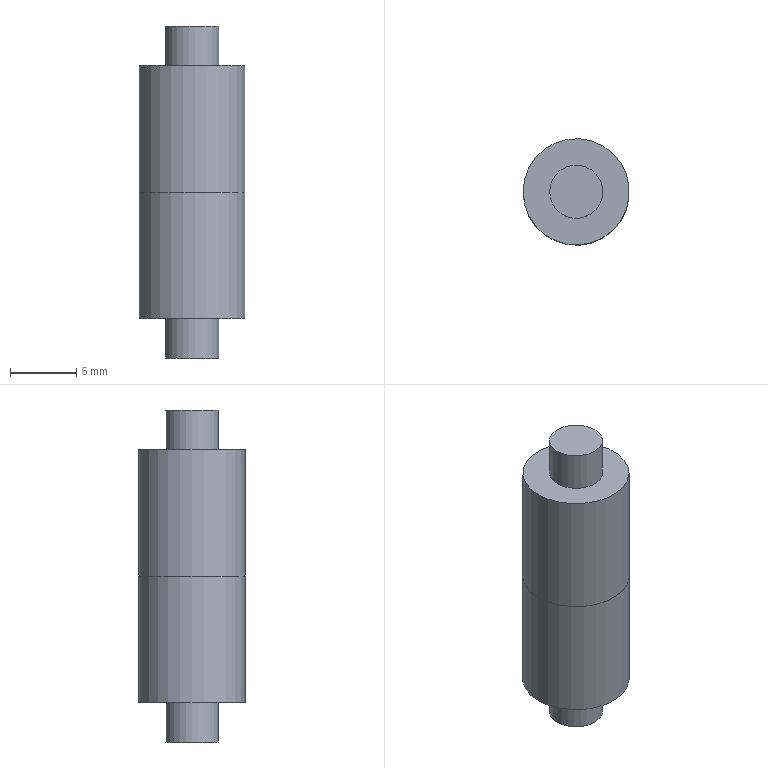Component | NX | MODEL5 | 2 solids | 10 faces | box 8 x 8 x 25 mm | volume 1030 mm3 | plane 6 | cylinder 4 | commonest cylinder face diameters 8 x2 4 x2
STEP:
#1=CARTESIAN_POINT('',(0.,0.,0.));
#2=DIRECTION('',(0.,0.,1.));
#3=DIRECTION('',(1.,0.,0.));
#4=AXIS2_PLACEMENT_3D('',#1,#2,#3);
#5=CARTESIAN_POINT('',(-1.53,2.589,6.));
#6=VERTEX_POINT('',#5);
#7=CARTESIAN_POINT('',(2.47,2.589,6.));
#8=DIRECTION('',(0.,0.,-1.));
#9=DIRECTION('',(-1.,0.,0.));
#10=AXIS2_PLACEMENT_3D('',#7,#8,#9);
#11=CIRCLE('',#10,4.);
#12=CARTESIAN_POINT('',(2.47,4.589,6.));
#13=DIRECTION('',(0.,0.,-1.));
#14=DIRECTION('',(-1.,0.,0.));
#15=AXIS2_PLACEMENT_3D('',#12,#13,#14);
#16=PLANE('',#15);
#17=CARTESIAN_POINT('',(0.,-2.));
#18=DIRECTION('',(1.,0.));
#19=AXIS2_PLACEMENT_2D('',#17,#18);
#20=CIRCLE('',#19,4.);
#21=(GEOMETRIC_REPRESENTATION_CONTEXT(2)PARAMETRIC_REPRESENTATION_CONTEXT()REPRESENTATION_CONTEXT('',''));
#22=DEFINITIONAL_REPRESENTATION('',(#20),#21);
#23=PCURVE('',#16,#22);
#24=CARTESIAN_POINT('',(2.47,2.589,3.));
#25=DIRECTION('',(0.,0.,-1.));
#26=DIRECTION('',(-1.,0.,0.));
#27=AXIS2_PLACEMENT_3D('',#24,#25,#26);
#28=CYLINDRICAL_SURFACE('',#27,4.);
#29=CARTESIAN_POINT('',(0.,-3.));
#30=DIRECTION('',(1.,0.));
#31=VECTOR('',#30,1.);
#32=LINE('',#29,#31);
#33=(GEOMETRIC_REPRESENTATION_CONTEXT(2)PARAMETRIC_REPRESENTATION_CONTEXT()REPRESENTATION_CONTEXT('',''));
#34=DEFINITIONAL_REPRESENTATION('',(#32),#33);
#35=PCURVE('',#28,#34);
#36=SURFACE_CURVE('',#11,(#23,#35),.PCURVE_S1.);
#37=EDGE_CURVE('',#6,#6,#36,.T.);
#38=ORIENTED_EDGE('',*,*,#37,.T.);
#39=EDGE_LOOP('',(#38));
#40=FACE_BOUND('',#39,.T.);
#41=CARTESIAN_POINT('',(0.4703,2.589,6.));
#42=VERTEX_POINT('',#41);
#43=CARTESIAN_POINT('',(2.47,2.589,6.));
#44=DIRECTION('',(0.,0.,-1.));
#45=DIRECTION('',(-1.,0.,0.));
#46=AXIS2_PLACEMENT_3D('',#43,#44,#45);
#47=CIRCLE('',#46,2.);
#48=CARTESIAN_POINT('',(0.,-2.));
#49=DIRECTION('',(1.,0.));
#50=AXIS2_PLACEMENT_2D('',#48,#49);
#51=CIRCLE('',#50,2.);
#52=(GEOMETRIC_REPRESENTATION_CONTEXT(2)PARAMETRIC_REPRESENTATION_CONTEXT()REPRESENTATION_CONTEXT('',''));
#53=DEFINITIONAL_REPRESENTATION('',(#51),#52);
#54=PCURVE('',#16,#53);
#55=CARTESIAN_POINT('',(2.47,2.589,3.));
#56=DIRECTION('',(0.,0.,-1.));
#57=DIRECTION('',(-1.,0.,0.));
#58=AXIS2_PLACEMENT_3D('',#55,#56,#57);
#59=CYLINDRICAL_SURFACE('',#58,2.);
#60=CARTESIAN_POINT('',(0.,-3.));
#61=DIRECTION('',(1.,0.));
#62=VECTOR('',#61,1.);
#63=LINE('',#60,#62);
#64=(GEOMETRIC_REPRESENTATION_CONTEXT(2)PARAMETRIC_REPRESENTATION_CONTEXT()REPRESENTATION_CONTEXT('',''));
#65=DEFINITIONAL_REPRESENTATION('',(#63),#64);
#66=PCURVE('',#59,#65);
#67=SURFACE_CURVE('',#47,(#54,#66),.PCURVE_S1.);
#68=EDGE_CURVE('',#42,#42,#67,.T.);
#69=ORIENTED_EDGE('',*,*,#68,.F.);
#70=EDGE_LOOP('',(#69));
#71=FACE_BOUND('',#70,.T.);
#72=ADVANCED_FACE('',(#40,#71),#16,.T.);
#73=CARTESIAN_POINT('',(-1.53,2.589,15.5));
#74=VERTEX_POINT('',#73);
#75=CARTESIAN_POINT('',(2.47,2.589,15.5));
#76=DIRECTION('',(0.,0.,-1.));
#77=DIRECTION('',(-1.,0.,0.));
#78=AXIS2_PLACEMENT_3D('',#75,#76,#77);
#79=CIRCLE('',#78,4.);
#80=CARTESIAN_POINT('',(0.,-12.5));
#81=DIRECTION('',(1.,0.));
#82=VECTOR('',#81,1.);
#83=LINE('',#80,#82);
#84=(GEOMETRIC_REPRESENTATION_CONTEXT(2)PARAMETRIC_REPRESENTATION_CONTEXT()REPRESENTATION_CONTEXT('',''));
#85=DEFINITIONAL_REPRESENTATION('',(#83),#84);
#86=PCURVE('',#28,#85);
#87=CARTESIAN_POINT('',(2.47,6.589,15.5));
#88=DIRECTION('',(0.,0.,1.));
#89=DIRECTION('',(1.,0.,0.));
#90=AXIS2_PLACEMENT_3D('',#87,#88,#89);
#91=PLANE('',#90);
#92=CARTESIAN_POINT('',(-4.,-4.));
#93=CARTESIAN_POINT('',(-4.,2.928));
#94=CARTESIAN_POINT('',(2.,-0.5359));
#95=CARTESIAN_POINT('',(8.,-4.));
#96=CARTESIAN_POINT('',(2.,-7.464));
#97=CARTESIAN_POINT('',(-4.,-10.928));
#98=CARTESIAN_POINT('',(-4.,-4.));
#99=(BOUNDED_CURVE()B_SPLINE_CURVE(2,(#92,#93,#94,#95,#96,#97,#98),.UNSPECIFIED.,.T.,.F.)B_SPLINE_CURVE_WITH_KNOTS((1,2,2,2,2,1),(-2.094,0.,2.094,4.189,6.283,8.378),.UNSPECIFIED.)CURVE()GEOMETRIC_REPRESENTATION_ITEM()RATIONAL_B_SPLINE_CURVE((1.,0.5,1.,0.5,1.,0.5,1.))REPRESENTATION_ITEM(''));
#100=(GEOMETRIC_REPRESENTATION_CONTEXT(2)PARAMETRIC_REPRESENTATION_CONTEXT()REPRESENTATION_CONTEXT('',''));
#101=DEFINITIONAL_REPRESENTATION('',(#99),#100);
#102=PCURVE('',#91,#101);
#103=SURFACE_CURVE('',#79,(#86,#102),.PCURVE_S1.);
#104=EDGE_CURVE('',#74,#74,#103,.T.);
#105=ORIENTED_EDGE('',*,*,#104,.T.);
#106=CARTESIAN_POINT('',(-1.53,2.589,15.5));
#107=CARTESIAN_POINT('',(-1.53,2.589,6.));
#108=B_SPLINE_CURVE_WITH_KNOTS('',1,(#106,#107),.UNSPECIFIED.,.F.,.F.,(2,2),(-12.5,-3.),.PIECEWISE_BEZIER_KNOTS.);
#109=CARTESIAN_POINT('',(6.283,0.));
#110=DIRECTION('',(0.,1.));
#111=VECTOR('',#110,1.);
#112=LINE('',#109,#111);
#113=(GEOMETRIC_REPRESENTATION_CONTEXT(2)PARAMETRIC_REPRESENTATION_CONTEXT()REPRESENTATION_CONTEXT('',''));
#114=DEFINITIONAL_REPRESENTATION('',(#112),#113);
#115=PCURVE('',#28,#114);
#116=CARTESIAN_POINT('',(0.,0.));
#117=DIRECTION('',(0.,1.));
#118=VECTOR('',#117,1.);
#119=LINE('',#116,#118);
#120=(GEOMETRIC_REPRESENTATION_CONTEXT(2)PARAMETRIC_REPRESENTATION_CONTEXT()REPRESENTATION_CONTEXT('',''));
#121=DEFINITIONAL_REPRESENTATION('',(#119),#120);
#122=PCURVE('',#28,#121);
#123=SEAM_CURVE('',#108,(#115,#122),.PCURVE_S1.);
#124=EDGE_CURVE('',#74,#6,#123,.T.);
#125=ORIENTED_EDGE('',*,*,#124,.T.);
#126=ORIENTED_EDGE('',*,*,#37,.F.);
#127=ORIENTED_EDGE('',*,*,#124,.F.);
#128=EDGE_LOOP('',(#105,#125,#126,#127));
#129=FACE_BOUND('',#128,.T.);
#130=ADVANCED_FACE('',(#129),#28,.T.);
#131=ORIENTED_EDGE('',*,*,#104,.F.);
#132=EDGE_LOOP('',(#131));
#133=FACE_BOUND('',#132,.T.);
#134=ADVANCED_FACE('',(#133),#91,.T.);
#135=CARTESIAN_POINT('',(0.4703,2.589,3.));
#136=VERTEX_POINT('',#135);
#137=CARTESIAN_POINT('',(2.47,2.589,3.));
#138=DIRECTION('',(0.,0.,-1.));
#139=DIRECTION('',(-1.,0.,0.));
#140=AXIS2_PLACEMENT_3D('',#137,#138,#139);
#141=CIRCLE('',#140,2.);
#142=CARTESIAN_POINT('',(2.47,2.589,3.));
#143=DIRECTION('',(0.,0.,-1.));
#144=DIRECTION('',(-1.,0.,0.));
#145=AXIS2_PLACEMENT_3D('',#142,#143,#144);
#146=PLANE('',#145);
#147=CARTESIAN_POINT('',(0.,0.));
#148=DIRECTION('',(1.,0.));
#149=AXIS2_PLACEMENT_2D('',#147,#148);
#150=CIRCLE('',#149,2.);
#151=(GEOMETRIC_REPRESENTATION_CONTEXT(2)PARAMETRIC_REPRESENTATION_CONTEXT()REPRESENTATION_CONTEXT('',''));
#152=DEFINITIONAL_REPRESENTATION('',(#150),#151);
#153=PCURVE('',#146,#152);
#154=CARTESIAN_POINT('',(0.,0.));
#155=DIRECTION('',(1.,0.));
#156=VECTOR('',#155,1.);
#157=LINE('',#154,#156);
#158=(GEOMETRIC_REPRESENTATION_CONTEXT(2)PARAMETRIC_REPRESENTATION_CONTEXT()REPRESENTATION_CONTEXT('',''));
#159=DEFINITIONAL_REPRESENTATION('',(#157),#158);
#160=PCURVE('',#59,#159);
#161=SURFACE_CURVE('',#141,(#153,#160),.PCURVE_S1.);
#162=EDGE_CURVE('',#136,#136,#161,.T.);
#163=ORIENTED_EDGE('',*,*,#162,.T.);
#164=EDGE_LOOP('',(#163));
#165=FACE_BOUND('',#164,.T.);
#166=ADVANCED_FACE('',(#165),#146,.T.);
#167=ORIENTED_EDGE('',*,*,#68,.T.);
#168=CARTESIAN_POINT('',(0.4703,2.589,6.));
#169=CARTESIAN_POINT('',(0.4703,2.589,3.));
#170=B_SPLINE_CURVE_WITH_KNOTS('',1,(#168,#169),.UNSPECIFIED.,.F.,.F.,(2,2),(-3.,0.),.PIECEWISE_BEZIER_KNOTS.);
#171=CARTESIAN_POINT('',(6.283,0.));
#172=DIRECTION('',(0.,1.));
#173=VECTOR('',#172,1.);
#174=LINE('',#171,#173);
#175=(GEOMETRIC_REPRESENTATION_CONTEXT(2)PARAMETRIC_REPRESENTATION_CONTEXT()REPRESENTATION_CONTEXT('',''));
#176=DEFINITIONAL_REPRESENTATION('',(#174),#175);
#177=PCURVE('',#59,#176);
#178=CARTESIAN_POINT('',(0.,0.));
#179=DIRECTION('',(0.,1.));
#180=VECTOR('',#179,1.);
#181=LINE('',#178,#180);
#182=(GEOMETRIC_REPRESENTATION_CONTEXT(2)PARAMETRIC_REPRESENTATION_CONTEXT()REPRESENTATION_CONTEXT('',''));
#183=DEFINITIONAL_REPRESENTATION('',(#181),#182);
#184=PCURVE('',#59,#183);
#185=SEAM_CURVE('',#170,(#177,#184),.PCURVE_S1.);
#186=EDGE_CURVE('',#42,#136,#185,.T.);
#187=ORIENTED_EDGE('',*,*,#186,.T.);
#188=ORIENTED_EDGE('',*,*,#162,.F.);
#189=ORIENTED_EDGE('',*,*,#186,.F.);
#190=EDGE_LOOP('',(#167,#187,#188,#189));
#191=FACE_BOUND('',#190,.T.);
#192=ADVANCED_FACE('',(#191),#59,.T.);
#193=CLOSED_SHELL('',(#72,#130,#134,#166,#192));
#194=MANIFOLD_SOLID_BREP('',#193);
#195=(LENGTH_UNIT()NAMED_UNIT(*)SI_UNIT(.MILLI.,.METRE.));
#196=UNCERTAINTY_MEASURE_WITH_UNIT(LENGTH_MEASURE(0.00001),#195,'','');
#197=(NAMED_UNIT(*)PLANE_ANGLE_UNIT()SI_UNIT($,.RADIAN.));
#198=(NAMED_UNIT(*)SI_UNIT($,.STERADIAN.)SOLID_ANGLE_UNIT());
#199=(GEOMETRIC_REPRESENTATION_CONTEXT(3)GLOBAL_UNCERTAINTY_ASSIGNED_CONTEXT((#196))GLOBAL_UNIT_ASSIGNED_CONTEXT((#195,#197,#198))REPRESENTATION_CONTEXT('',''));
#200=ADVANCED_BREP_SHAPE_REPRESENTATION('',(#4,#194),#199);
#201=CARTESIAN_POINT('',(0.,0.,0.));
#202=DIRECTION('',(0.,0.,1.));
#203=DIRECTION('',(1.,0.,0.));
#204=AXIS2_PLACEMENT_3D('',#201,#202,#203);
#205=CARTESIAN_POINT('',(0.,0.,0.));
#206=DIRECTION('',(0.,0.,1.));
#207=DIRECTION('',(1.,0.,0.));
#208=AXIS2_PLACEMENT_3D('',#205,#206,#207);
#209=(LENGTH_UNIT()NAMED_UNIT(*)SI_UNIT(.MILLI.,.METRE.));
#210=UNCERTAINTY_MEASURE_WITH_UNIT(LENGTH_MEASURE(0.00001),#209,'','');
#211=(NAMED_UNIT(*)PLANE_ANGLE_UNIT()SI_UNIT($,.RADIAN.));
#212=(NAMED_UNIT(*)SI_UNIT($,.STERADIAN.)SOLID_ANGLE_UNIT());
#213=(GEOMETRIC_REPRESENTATION_CONTEXT(3)GLOBAL_UNCERTAINTY_ASSIGNED_CONTEXT((#210))GLOBAL_UNIT_ASSIGNED_CONTEXT((#209,#211,#212))REPRESENTATION_CONTEXT('',''));
#214=SHAPE_REPRESENTATION('',(#4,#204,#208),#213);
#215=ITEM_DEFINED_TRANSFORMATION('','',#4,#204);
#216=(REPRESENTATION_RELATIONSHIP('','',#200,#214)REPRESENTATION_RELATIONSHIP_WITH_TRANSFORMATION(#215)SHAPE_REPRESENTATION_RELATIONSHIP());
#217=CARTESIAN_POINT('',(-1.53,2.589,25.));
#218=VERTEX_POINT('',#217);
#219=CARTESIAN_POINT('',(2.47,2.589,25.));
#220=DIRECTION('',(0.,0.,-1.));
#221=DIRECTION('',(-1.,0.,0.));
#222=AXIS2_PLACEMENT_3D('',#219,#220,#221);
#223=CIRCLE('',#222,4.);
#224=CARTESIAN_POINT('',(2.47,4.589,25.));
#225=DIRECTION('',(0.,0.,1.));
#226=DIRECTION('',(-1.,0.,0.));
#227=AXIS2_PLACEMENT_3D('',#224,#225,#226);
#228=PLANE('',#227);
#229=CARTESIAN_POINT('',(4.,2.));
#230=CARTESIAN_POINT('',(4.,-4.928));
#231=CARTESIAN_POINT('',(-2.,-1.464));
#232=CARTESIAN_POINT('',(-8.,2.));
#233=CARTESIAN_POINT('',(-2.,5.464));
#234=CARTESIAN_POINT('',(4.,8.928));
#235=CARTESIAN_POINT('',(4.,2.));
#236=(BOUNDED_CURVE()B_SPLINE_CURVE(2,(#229,#230,#231,#232,#233,#234,#235),.UNSPECIFIED.,.T.,.F.)B_SPLINE_CURVE_WITH_KNOTS((1,2,2,2,2,1),(-2.094,0.,2.094,4.189,6.283,8.378),.UNSPECIFIED.)CURVE()GEOMETRIC_REPRESENTATION_ITEM()RATIONAL_B_SPLINE_CURVE((1.,0.5,1.,0.5,1.,0.5,1.))REPRESENTATION_ITEM(''));
#237=(GEOMETRIC_REPRESENTATION_CONTEXT(2)PARAMETRIC_REPRESENTATION_CONTEXT()REPRESENTATION_CONTEXT('',''));
#238=DEFINITIONAL_REPRESENTATION('',(#236),#237);
#239=PCURVE('',#228,#238);
#240=CARTESIAN_POINT('',(2.47,2.589,28.));
#241=DIRECTION('',(0.,0.,1.));
#242=DIRECTION('',(-1.,0.,0.));
#243=AXIS2_PLACEMENT_3D('',#240,#241,#242);
#244=CYLINDRICAL_SURFACE('',#243,4.);
#245=CARTESIAN_POINT('',(6.283,-3.));
#246=DIRECTION('',(-1.,0.));
#247=VECTOR('',#246,1.);
#248=LINE('',#245,#247);
#249=(GEOMETRIC_REPRESENTATION_CONTEXT(2)PARAMETRIC_REPRESENTATION_CONTEXT()REPRESENTATION_CONTEXT('',''));
#250=DEFINITIONAL_REPRESENTATION('',(#248),#249);
#251=PCURVE('',#244,#250);
#252=SURFACE_CURVE('',#223,(#239,#251),.PCURVE_S1.);
#253=EDGE_CURVE('',#218,#218,#252,.T.);
#254=ORIENTED_EDGE('',*,*,#253,.F.);
#255=EDGE_LOOP('',(#254));
#256=FACE_BOUND('',#255,.T.);
#257=CARTESIAN_POINT('',(0.4703,2.589,25.));
#258=VERTEX_POINT('',#257);
#259=CARTESIAN_POINT('',(2.47,2.589,25.));
#260=DIRECTION('',(0.,0.,-1.));
#261=DIRECTION('',(-1.,0.,0.));
#262=AXIS2_PLACEMENT_3D('',#259,#260,#261);
#263=CIRCLE('',#262,2.);
#264=CARTESIAN_POINT('',(2.,2.));
#265=CARTESIAN_POINT('',(2.,-1.464));
#266=CARTESIAN_POINT('',(-1.,0.2679));
#267=CARTESIAN_POINT('',(-4.,2.));
#268=CARTESIAN_POINT('',(-1.,3.732));
#269=CARTESIAN_POINT('',(2.,5.464));
#270=CARTESIAN_POINT('',(2.,2.));
#271=(BOUNDED_CURVE()B_SPLINE_CURVE(2,(#264,#265,#266,#267,#268,#269,#270),.UNSPECIFIED.,.T.,.F.)B_SPLINE_CURVE_WITH_KNOTS((1,2,2,2,2,1),(-2.094,0.,2.094,4.189,6.283,8.378),.UNSPECIFIED.)CURVE()GEOMETRIC_REPRESENTATION_ITEM()RATIONAL_B_SPLINE_CURVE((1.,0.5,1.,0.5,1.,0.5,1.))REPRESENTATION_ITEM(''));
#272=(GEOMETRIC_REPRESENTATION_CONTEXT(2)PARAMETRIC_REPRESENTATION_CONTEXT()REPRESENTATION_CONTEXT('',''));
#273=DEFINITIONAL_REPRESENTATION('',(#271),#272);
#274=PCURVE('',#228,#273);
#275=CARTESIAN_POINT('',(2.47,2.589,28.));
#276=DIRECTION('',(0.,0.,1.));
#277=DIRECTION('',(-1.,0.,0.));
#278=AXIS2_PLACEMENT_3D('',#275,#276,#277);
#279=CYLINDRICAL_SURFACE('',#278,2.);
#280=CARTESIAN_POINT('',(6.283,-3.));
#281=DIRECTION('',(-1.,0.));
#282=VECTOR('',#281,1.);
#283=LINE('',#280,#282);
#284=(GEOMETRIC_REPRESENTATION_CONTEXT(2)PARAMETRIC_REPRESENTATION_CONTEXT()REPRESENTATION_CONTEXT('',''));
#285=DEFINITIONAL_REPRESENTATION('',(#283),#284);
#286=PCURVE('',#279,#285);
#287=SURFACE_CURVE('',#263,(#274,#286),.PCURVE_S1.);
#288=EDGE_CURVE('',#258,#258,#287,.T.);
#289=ORIENTED_EDGE('',*,*,#288,.T.);
#290=EDGE_LOOP('',(#289));
#291=FACE_BOUND('',#290,.T.);
#292=ADVANCED_FACE('',(#256,#291),#228,.T.);
#293=CARTESIAN_POINT('',(-1.53,2.589,15.5));
#294=VERTEX_POINT('',#293);
#295=CARTESIAN_POINT('',(2.47,2.589,15.5));
#296=DIRECTION('',(0.,0.,-1.));
#297=DIRECTION('',(-1.,0.,0.));
#298=AXIS2_PLACEMENT_3D('',#295,#296,#297);
#299=CIRCLE('',#298,4.);
#300=CARTESIAN_POINT('',(6.283,-12.5));
#301=DIRECTION('',(-1.,0.));
#302=VECTOR('',#301,1.);
#303=LINE('',#300,#302);
#304=(GEOMETRIC_REPRESENTATION_CONTEXT(2)PARAMETRIC_REPRESENTATION_CONTEXT()REPRESENTATION_CONTEXT('',''));
#305=DEFINITIONAL_REPRESENTATION('',(#303),#304);
#306=PCURVE('',#244,#305);
#307=CARTESIAN_POINT('',(2.47,6.589,15.5));
#308=DIRECTION('',(0.,0.,-1.));
#309=DIRECTION('',(1.,0.,0.));
#310=AXIS2_PLACEMENT_3D('',#307,#308,#309);
#311=PLANE('',#310);
#312=CARTESIAN_POINT('',(0.,4.));
#313=DIRECTION('',(-1.,0.));
#314=AXIS2_PLACEMENT_2D('',#312,#313);
#315=CIRCLE('',#314,4.);
#316=(GEOMETRIC_REPRESENTATION_CONTEXT(2)PARAMETRIC_REPRESENTATION_CONTEXT()REPRESENTATION_CONTEXT('',''));
#317=DEFINITIONAL_REPRESENTATION('',(#315),#316);
#318=PCURVE('',#311,#317);
#319=SURFACE_CURVE('',#299,(#306,#318),.PCURVE_S1.);
#320=EDGE_CURVE('',#294,#294,#319,.T.);
#321=ORIENTED_EDGE('',*,*,#320,.F.);
#322=CARTESIAN_POINT('',(-1.53,2.589,15.5));
#323=CARTESIAN_POINT('',(-1.53,2.589,25.));
#324=B_SPLINE_CURVE_WITH_KNOTS('',1,(#322,#323),.UNSPECIFIED.,.F.,.F.,(2,2),(-12.5,-3.),.PIECEWISE_BEZIER_KNOTS.);
#325=CARTESIAN_POINT('',(6.283,0.));
#326=DIRECTION('',(0.,1.));
#327=VECTOR('',#326,1.);
#328=LINE('',#325,#327);
#329=(GEOMETRIC_REPRESENTATION_CONTEXT(2)PARAMETRIC_REPRESENTATION_CONTEXT()REPRESENTATION_CONTEXT('',''));
#330=DEFINITIONAL_REPRESENTATION('',(#328),#329);
#331=PCURVE('',#244,#330);
#332=CARTESIAN_POINT('',(0.,0.));
#333=DIRECTION('',(0.,1.));
#334=VECTOR('',#333,1.);
#335=LINE('',#332,#334);
#336=(GEOMETRIC_REPRESENTATION_CONTEXT(2)PARAMETRIC_REPRESENTATION_CONTEXT()REPRESENTATION_CONTEXT('',''));
#337=DEFINITIONAL_REPRESENTATION('',(#335),#336);
#338=PCURVE('',#244,#337);
#339=SEAM_CURVE('',#324,(#331,#338),.PCURVE_S1.);
#340=EDGE_CURVE('',#294,#218,#339,.T.);
#341=ORIENTED_EDGE('',*,*,#340,.T.);
#342=ORIENTED_EDGE('',*,*,#253,.T.);
#343=ORIENTED_EDGE('',*,*,#340,.F.);
#344=EDGE_LOOP('',(#321,#341,#342,#343));
#345=FACE_BOUND('',#344,.T.);
#346=ADVANCED_FACE('',(#345),#244,.T.);
#347=ORIENTED_EDGE('',*,*,#320,.T.);
#348=EDGE_LOOP('',(#347));
#349=FACE_BOUND('',#348,.T.);
#350=ADVANCED_FACE('',(#349),#311,.T.);
#351=CARTESIAN_POINT('',(0.4703,2.589,28.));
#352=VERTEX_POINT('',#351);
#353=CARTESIAN_POINT('',(2.47,2.589,28.));
#354=DIRECTION('',(0.,0.,-1.));
#355=DIRECTION('',(-1.,0.,0.));
#356=AXIS2_PLACEMENT_3D('',#353,#354,#355);
#357=CIRCLE('',#356,2.);
#358=CARTESIAN_POINT('',(2.47,2.589,28.));
#359=DIRECTION('',(0.,0.,1.));
#360=DIRECTION('',(-1.,0.,0.));
#361=AXIS2_PLACEMENT_3D('',#358,#359,#360);
#362=PLANE('',#361);
#363=CARTESIAN_POINT('',(2.,0.));
#364=CARTESIAN_POINT('',(2.,-3.464));
#365=CARTESIAN_POINT('',(-1.,-1.732));
#366=CARTESIAN_POINT('',(-4.,-0.));
#367=CARTESIAN_POINT('',(-1.,1.732));
#368=CARTESIAN_POINT('',(2.,3.464));
#369=CARTESIAN_POINT('',(2.,0.));
#370=(BOUNDED_CURVE()B_SPLINE_CURVE(2,(#363,#364,#365,#366,#367,#368,#369),.UNSPECIFIED.,.T.,.F.)B_SPLINE_CURVE_WITH_KNOTS((1,2,2,2,2,1),(-2.094,0.,2.094,4.189,6.283,8.378),.UNSPECIFIED.)CURVE()GEOMETRIC_REPRESENTATION_ITEM()RATIONAL_B_SPLINE_CURVE((1.,0.5,1.,0.5,1.,0.5,1.))REPRESENTATION_ITEM(''));
#371=(GEOMETRIC_REPRESENTATION_CONTEXT(2)PARAMETRIC_REPRESENTATION_CONTEXT()REPRESENTATION_CONTEXT('',''));
#372=DEFINITIONAL_REPRESENTATION('',(#370),#371);
#373=PCURVE('',#362,#372);
#374=CARTESIAN_POINT('',(6.283,0.));
#375=DIRECTION('',(-1.,0.));
#376=VECTOR('',#375,1.);
#377=LINE('',#374,#376);
#378=(GEOMETRIC_REPRESENTATION_CONTEXT(2)PARAMETRIC_REPRESENTATION_CONTEXT()REPRESENTATION_CONTEXT('',''));
#379=DEFINITIONAL_REPRESENTATION('',(#377),#378);
#380=PCURVE('',#279,#379);
#381=SURFACE_CURVE('',#357,(#373,#380),.PCURVE_S1.);
#382=EDGE_CURVE('',#352,#352,#381,.T.);
#383=ORIENTED_EDGE('',*,*,#382,.F.);
#384=EDGE_LOOP('',(#383));
#385=FACE_BOUND('',#384,.T.);
#386=ADVANCED_FACE('',(#385),#362,.T.);
#387=ORIENTED_EDGE('',*,*,#288,.F.);
#388=CARTESIAN_POINT('',(0.4703,2.589,25.));
#389=CARTESIAN_POINT('',(0.4703,2.589,28.));
#390=B_SPLINE_CURVE_WITH_KNOTS('',1,(#388,#389),.UNSPECIFIED.,.F.,.F.,(2,2),(-3.,0.),.PIECEWISE_BEZIER_KNOTS.);
#391=CARTESIAN_POINT('',(6.283,0.));
#392=DIRECTION('',(0.,1.));
#393=VECTOR('',#392,1.);
#394=LINE('',#391,#393);
#395=(GEOMETRIC_REPRESENTATION_CONTEXT(2)PARAMETRIC_REPRESENTATION_CONTEXT()REPRESENTATION_CONTEXT('',''));
#396=DEFINITIONAL_REPRESENTATION('',(#394),#395);
#397=PCURVE('',#279,#396);
#398=CARTESIAN_POINT('',(0.,0.));
#399=DIRECTION('',(0.,1.));
#400=VECTOR('',#399,1.);
#401=LINE('',#398,#400);
#402=(GEOMETRIC_REPRESENTATION_CONTEXT(2)PARAMETRIC_REPRESENTATION_CONTEXT()REPRESENTATION_CONTEXT('',''));
#403=DEFINITIONAL_REPRESENTATION('',(#401),#402);
#404=PCURVE('',#279,#403);
#405=SEAM_CURVE('',#390,(#397,#404),.PCURVE_S1.);
#406=EDGE_CURVE('',#258,#352,#405,.T.);
#407=ORIENTED_EDGE('',*,*,#406,.T.);
#408=ORIENTED_EDGE('',*,*,#382,.T.);
#409=ORIENTED_EDGE('',*,*,#406,.F.);
#410=EDGE_LOOP('',(#387,#407,#408,#409));
#411=FACE_BOUND('',#410,.T.);
#412=ADVANCED_FACE('',(#411),#279,.T.);
#413=CLOSED_SHELL('',(#292,#346,#350,#386,#412));
#414=MANIFOLD_SOLID_BREP('',#413);
#415=(LENGTH_UNIT()NAMED_UNIT(*)SI_UNIT(.MILLI.,.METRE.));
#416=UNCERTAINTY_MEASURE_WITH_UNIT(LENGTH_MEASURE(0.00001),#415,'','');
#417=(NAMED_UNIT(*)PLANE_ANGLE_UNIT()SI_UNIT($,.RADIAN.));
#418=(NAMED_UNIT(*)SI_UNIT($,.STERADIAN.)SOLID_ANGLE_UNIT());
#419=(GEOMETRIC_REPRESENTATION_CONTEXT(3)GLOBAL_UNCERTAINTY_ASSIGNED_CONTEXT((#416))GLOBAL_UNIT_ASSIGNED_CONTEXT((#415,#417,#418))REPRESENTATION_CONTEXT('',''));
#420=ADVANCED_BREP_SHAPE_REPRESENTATION('',(#4,#414),#419);
#421=ITEM_DEFINED_TRANSFORMATION('','',#4,#208);
#422=(REPRESENTATION_RELATIONSHIP('','',#420,#214)REPRESENTATION_RELATIONSHIP_WITH_TRANSFORMATION(#421)SHAPE_REPRESENTATION_RELATIONSHIP());